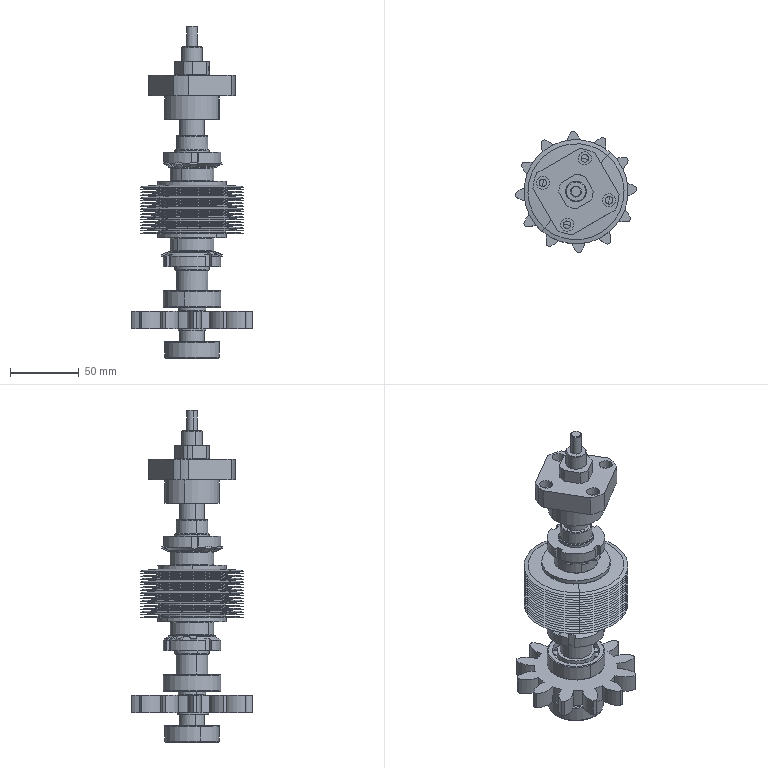Assembly | SolidWorks | mm | 49 component files | 49 solids | 914 faces | box 88.88 x 88.88 x 242 mm | volume 315904 mm3 | cylinder 344 | plane 220 | cone 161 | torus 111 | sphere 60 | spline 18 | commonest cylinder face diameters 25 x93 50 x38 30.48 x28 34 x14 60.322 x13 88.9 x12 32 x10 42 x10
Bill of materials:
0.8Gasket0 | 17 |  | Thin flat annular disc (plain washer-like ring) with a concentric round through-hole and square-cut edges.
108SingleEdgeBlade0 | 18 |  | Thin annular disc with a concentric central hole and a beveled/tapered outer rim; the hole is small relative to the outer diameter.
18A-typeShaftRetainingRing(GB-T894.1-1986)0 | 1 | 65Mn CH | Flat open split ring resembling an external retaining ring: an eccentric band with a radial gap and two widened lugs, each with a small round hole, at the open ends.
25RoundNutLockWasher(GB-T-858-1988)0 | 2 | 45 | Thin flat ring with several rectangular tabs projecting radially outward (six visible) and one rectangular tab projecting inward into the bore; outer tabs appear bent out of the ring plane.
3Gasket0 | 2 |  | Flat annular disc with concentric round through-hole, noticeably thicker than the other flat washers, with square edges.
6004DeepGrooveBallBearing(BG276-94)0 | 1 |  | Ball-bearing-like ring assembly: outer ring, inner ring and a single row of approximately 16 spheres between them, with open (unshielded) faces and slightly rounded edges.
6203OverrunningBearing0 | 1 | GCr15 | Ball-bearing-like ring assembly with a single row of spheres between outer and inner rings, with a rectangular notch in the outer ring and a small notch/step in the inner ring bore.
BladeDriveAxis0 | 1 |  | Long slender stepped cylindrical shaft with multiple diameter steps, a larger central body, circumferential grooves and small slot/keyway-like cuts near several shoulders and at one end.
FK15BallScrewSupportUnit(FixedSide)0 | 1 |  | Flanged housing/support block: a roughly square flange with clipped corners and four round through-holes, a central through-bore, a short cylindrical spigot on one side and a raised boss with two flat sides on the other, with small radial holes in the boss.
M25_1.5RoundNut(GB-T812-1988)0 | 2 |  | Short annular ring with several rectangular slots cut into its outer periphery and a chamfered outer edge on one face, resembling a slotted round nut.
Sleeve0 | 2 |  | Flat gear-like disc with 12 rounded, lobe-shaped radial teeth around a central hub and a round central through-hole, extruded to constant thickness.
spur gear_gb | 1 |  | Plain cylindrical sleeve/ring with thin wall relative to diameter, a moderate axial length, and small chamfers on the outer edges.
Mates:
1. coincident | 3Gasket0-1 face at (-15.093, -37.782, 215.255) dir (0, 0, -1) | Sleeve0-1 face at (-27.025, -27.888, 215.255) dir (0, 0, 1)
2. coincident | 25RoundNutLockWasher(GB-T-858-1988)0-1 face at (-15.093, -37.782, 205.255) dir (0, 0, 1) | Sleeve0-1 face at (-27.025, -27.888, 205.255) dir (0, 0, -1)
3. concentric | BladeDriveAxis0-2 face at (-15.093, -37.782, 127.655) dir (0, 0, -1) r 12.5 | 108SingleEdgeBlade0-5 face at (-15.093, -37.782, 209.455) dir (0, 0, 1) r 12.5
4. coincident | 25RoundNutLockWasher(GB-T-858-1988)0-1 face at (1.1, -32.606, 204.255) dir (0, 0, -1) | M25_1.5RoundNut(GB-T812-1988)0-2 face at (-7.474, -48.315, 204.255) dir (0, 0, 1)
5. concentric | BladeDriveAxis0-2 face at (-15.093, -37.782, 127.655) dir (0, 0, -1) r 9 | spur gear_gb-1 face at (-15.093, -37.782, 174.355) dir (0, 0, -1) r 9.525
6. coincident | BladeDriveAxis0-2 face at (-6.52, -35.042, 161.655) dir (0, 0, -1) | spur gear_gb-1 face at (-15.093, -37.782, 161.655) dir (0, 0, 1)
7. coincident | BladeDriveAxis0-2 face at (0.5844, -35.921, 149.055) dir (-0.3044, 0.9525, 0) | spur gear_gb-1 face at (-2.94, -37.047, 199.655) dir (-0.3044, 0.9525, 0)
8. coincident | spur gear_gb-1 face at (-15.093, -37.782, 148.955) dir (0, 0, -1) | 18A-typeShaftRetainingRing(GB-T894.1-1986)0-2 face at (-15.093, -37.782, 148.955) dir (0, 0, 1)
9. concentric | BladeDriveAxis0-2 face at (-15.093, -37.782, 127.655) dir (0, 0, -1) r 9 | 18A-typeShaftRetainingRing(GB-T894.1-1986)0-2 face at (-15.093, -37.782, 148.955) dir (0, 0, -1) r 8.5
10. concentric | BladeDriveAxis0-2 face at (-15.093, -37.782, 127.655) dir (0, 0, -1) r 8.5 | 6203OverrunningBearing0-1 face at (-15.093, -37.782, 155.11) dir (0, 0, 1) r 8.5
11. coincident | BladeDriveAxis0-2 face at (-6.997, -35.194, 139.655) dir (0, 0, -1) | 6203OverrunningBearing0-1 face at (-18.848, -26.032, 139.655) dir (0, 0, 1)
12. concentric | Sleeve0-1 face at (-15.093, -37.782, 243.036) dir (0, 0, 1) r 16 | BladeDriveAxis0-2 face at (-15.093, -37.782, 127.655) dir (0, 0, -1) r 12.5
13. concentric | 3Gasket0-1 face at (-15.093, -37.782, 218.255) dir (0, 0, -1) r 25 | BladeDriveAxis0-2 face at (-15.093, -37.782, 127.655) dir (0, 0, -1) r 12.5
14. concentric | M25_1.5RoundNut(GB-T812-1988)0-2 face at (-15.093, -37.782, 237.987) dir (0, 0, 1) r 21 | BladeDriveAxis0-2 face at (-15.093, -37.782, 127.655) dir (0, 0, -1) r 12.5
15. concentric | 25RoundNutLockWasher(GB-T-858-1988)0-1 face at (-15.093, -37.782, 194.255) dir (0, 0, 1) r 12.75 | BladeDriveAxis0-2 face at (-15.093, -37.782, 127.655) dir (0, 0, -1) r 12.5
16. concentric | BladeDriveAxis0-2 face at (-15.093, -37.782, 127.655) dir (0, 0, -1) r 10 | 6004DeepGrooveBallBearing(BG276-94)0-2 face at (-15.093, -37.782, 170.655) dir (0, 0, 1) r 21
17. coincident | BladeDriveAxis0-2 face at (-5.568, -34.737, 176.655) dir (0, 0, -1) | 6004DeepGrooveBallBearing(BG276-94)0-2 face at (-1.908, -41.371, 176.655) dir (0, 0, 1)
18. coincident | 3Gasket0-1 face at (-15.093, -37.782, 218.255) dir (0, 0, 1) | 108SingleEdgeBlade0-5 face at (-18.873, -34.508, 218.255) dir (0, 0, -1)
19. concentric | BladeDriveAxis0-2 face at (-15.093, -37.782, 127.655) dir (0, 0, -1) r 12.5 | 0.8Gasket0-3 face at (-15.093, -37.782, 220.255) dir (0, 0, -1) r 12.5
20. coincident | 108SingleEdgeBlade0-5 face at (-33.992, -21.416, 219.455) dir (0, 0, 1) | 0.8Gasket0-3 face at (-15.093, -37.782, 219.455) dir (0, 0, -1)
21. concentric | BladeDriveAxis0-2 face at (-15.093, -37.782, 127.655) dir (0, 0, -1) r 12.5 | Sleeve0-3 face at (-15.093, -37.782, 294.236) dir (0, 0, 1) r 16
22. concentric | 25RoundNutLockWasher(GB-T-858-1988)0-4 face at (-15.093, -37.782, 277.455) dir (0, 0, -1) r 12.75 | BladeDriveAxis0-2 face at (-15.093, -37.782, 127.655) dir (0, 0, -1) r 12.5
23. coincident | 25RoundNutLockWasher(GB-T-858-1988)0-4 face at (-15.093, -37.782, 266.455) dir (0, 0, -1) | Sleeve0-3 face at (-28.508, -30.016, 266.455) dir (0, 0, 1)
24. concentric | BladeDriveAxis0-2 face at (-15.093, -37.782, 127.655) dir (0, 0, -1) r 12.5 | M25_1.5RoundNut(GB-T812-1988)0-3 face at (-15.093, -37.782, 233.724) dir (0, 0, -1) r 12.5
25. coincident | 25RoundNutLockWasher(GB-T-858-1988)0-4 face at (1.1, -32.606, 267.455) dir (0, 0, 1) | M25_1.5RoundNut(GB-T812-1988)0-3 face at (-16.359, -24.843, 267.455) dir (0, 0, -1)
26. coincident | 108SingleEdgeBlade0-38 face at (-33.992, -21.416, 253.455) dir (0, 0, 1) | 3Gasket0-4 face at (-15.093, -37.782, 253.455) dir (0, 0, -1)
27. concentric | Sleeve0-3 face at (-15.093, -37.782, 294.236) dir (0, 0, 1) r 16 | 3Gasket0-4 face at (-15.093, -37.782, 256.455) dir (0, 0, -1) r 25
28. coincident | Sleeve0-3 face at (-28.508, -30.016, 256.455) dir (0, 0, -1) | 3Gasket0-4 face at (-15.093, -37.782, 256.455) dir (0, 0, 1)
29. distance | 6004DeepGrooveBallBearing(BG276-94)0-2 face at (4.591, -43.14, 176.655) dir (0, 0, 1) | 108SingleEdgeBlade0-5 face at (-18.873, -34.508, 218.255) dir (0, 0, -1)
30. concentric | BladeDriveAxis0-2 face at (-15.093, -37.782, 127.655) dir (0, 0, -1) r 7.5 | FK15BallScrewSupportUnit(FixedSide)0-1 face at (-15.093, -37.782, 368.655) dir (0, 0, -1) r 20
31. coincident | BladeDriveAxis0-2 face at (-6.52, -35.042, 307.655) dir (0, 0, 1) | FK15BallScrewSupportUnit(FixedSide)0-1 face at (-12.417, -27.68, 307.655) dir (0, 0, -1)
32. coincident | 108SingleEdgeBlade0-38 face at (-33.992, -21.416, 253.455) dir (0, 0, 1) | 3Gasket0-4 face at (-15.093, -37.782, 253.455) dir (0, 0, -1)